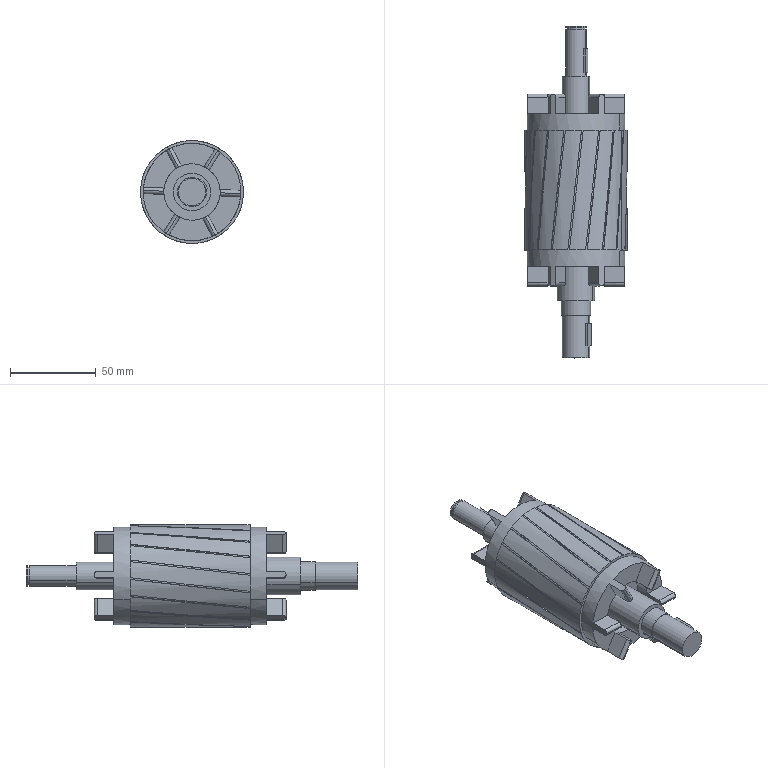Component | SolidWorks | Rotor-1 | 1 solid | 177 faces | box 60 x 193.75 x 60 mm | volume 265279 mm3 | cylinder 66 | plane 57 | spline 54 | commonest cylinder face diameters 3.75 x24 60 x20 16 x4 12 x4 33 x4 57 x4 17 x2 11 x2